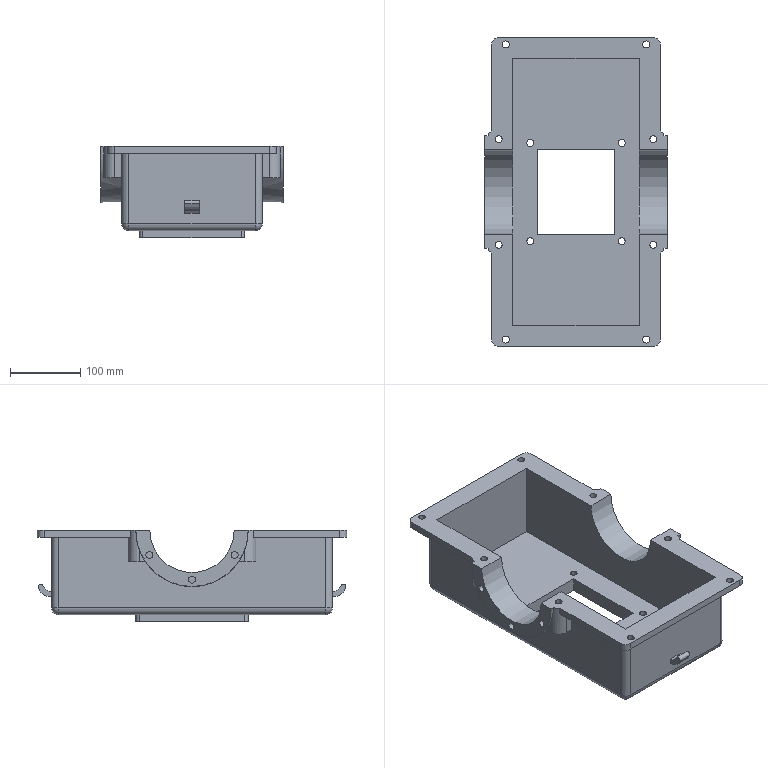Component | SolidWorks | WormGearReducerUpperCasing-1 | 1 solid | 124 faces | volume 2382449 mm3 | cylinder 67 | plane 53 | sphere 4 | commonest cylinder face diameters 10 x40 20 x12 32 x4 7.5 x3 160 x2 120 x2 25 x2 40 x2